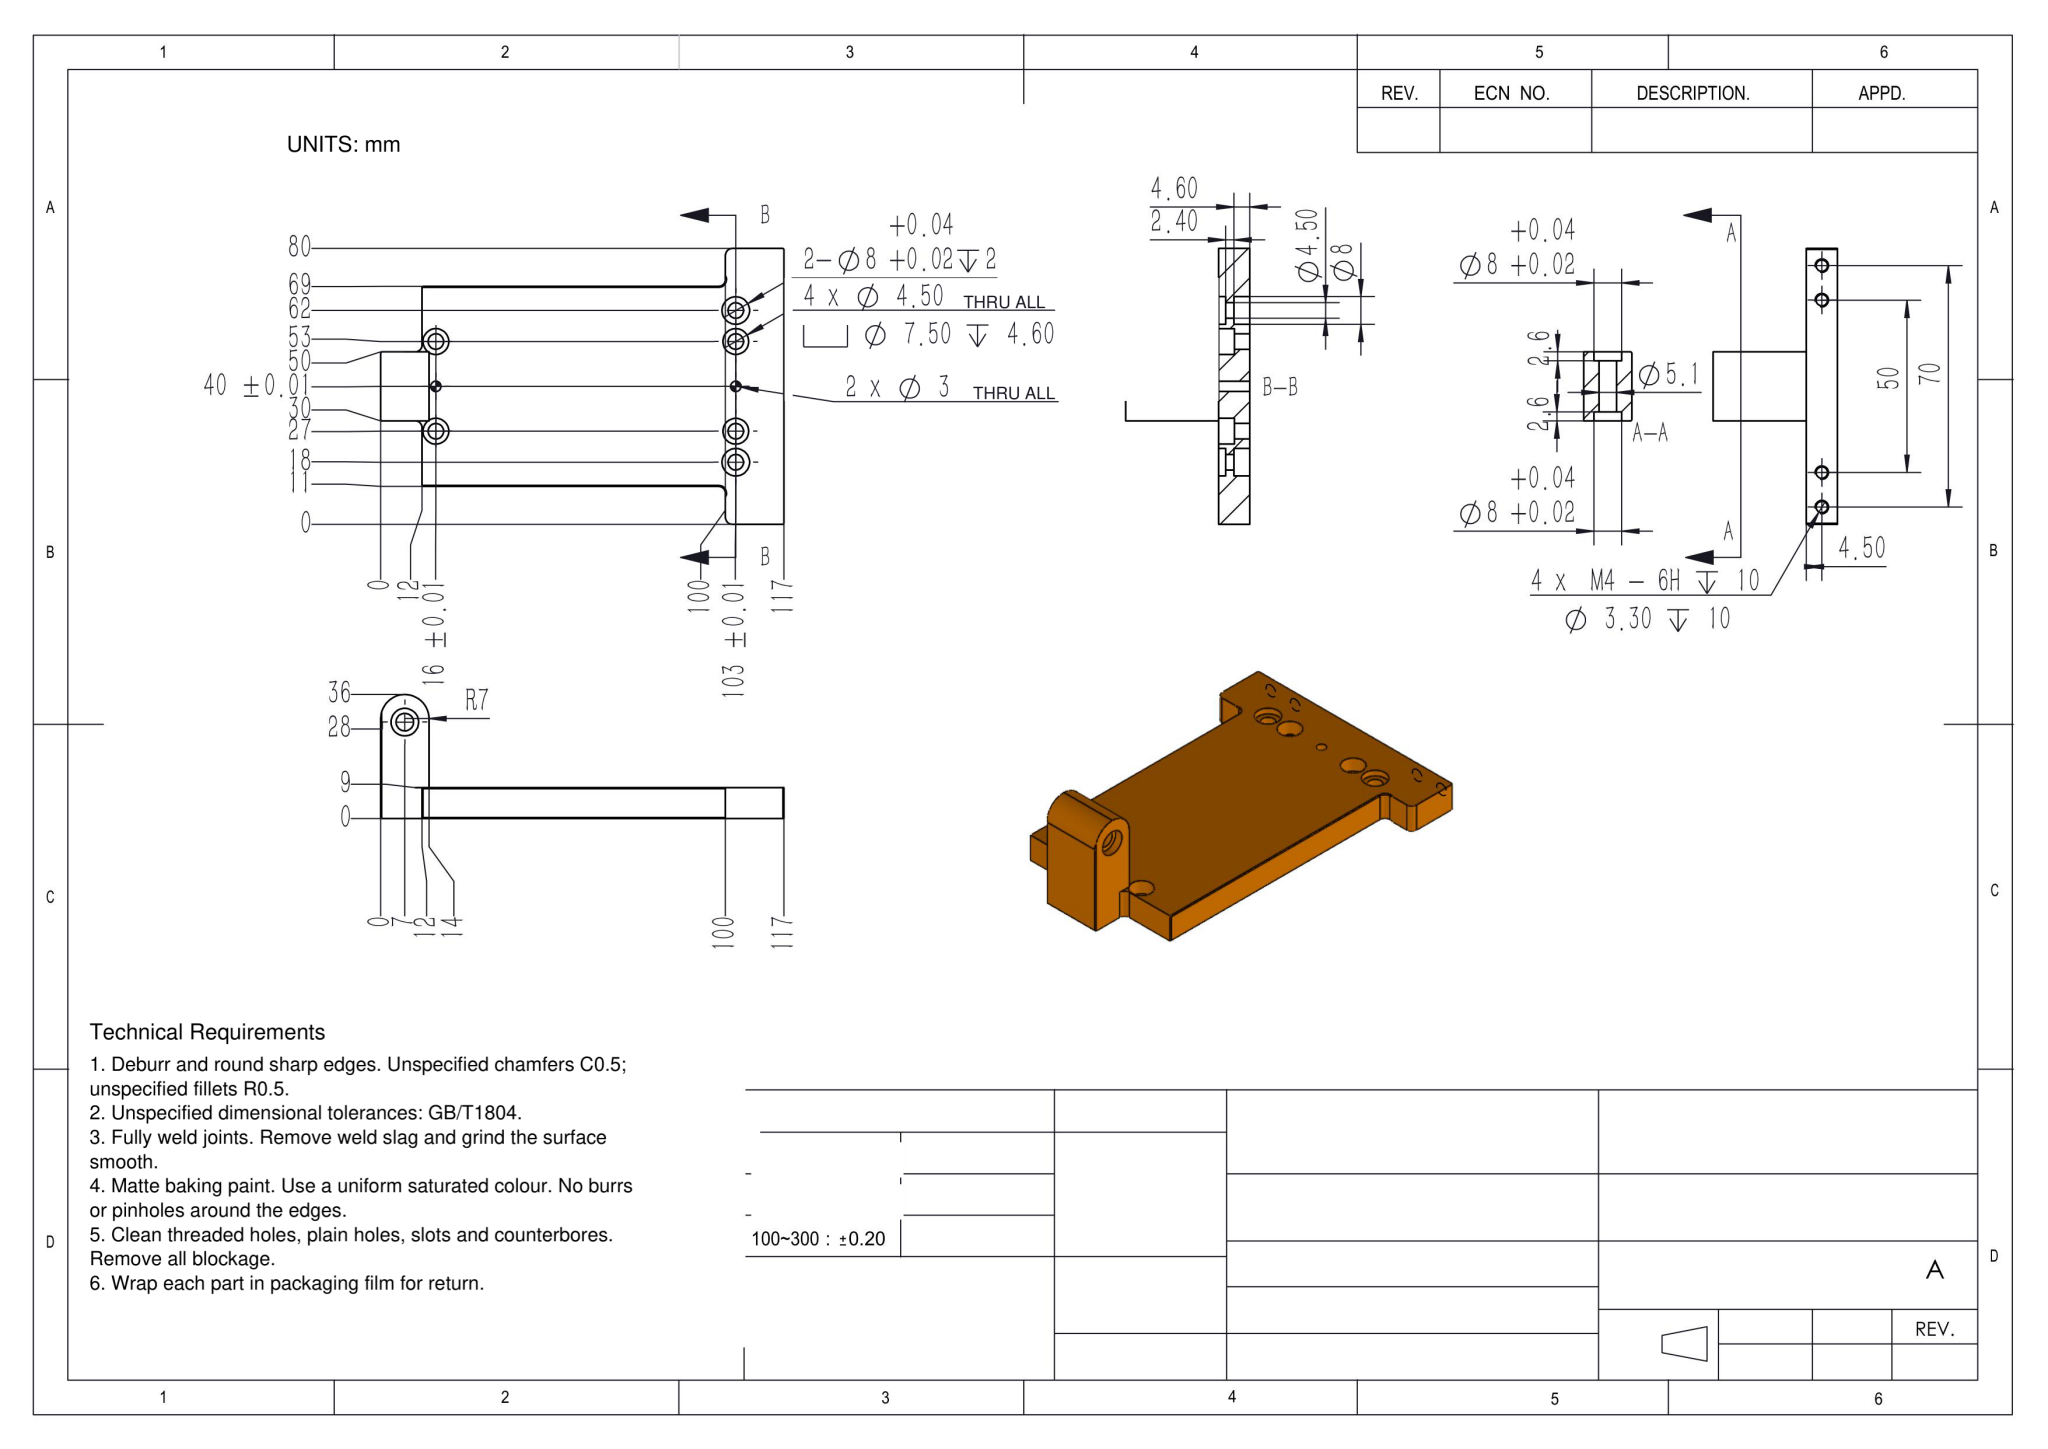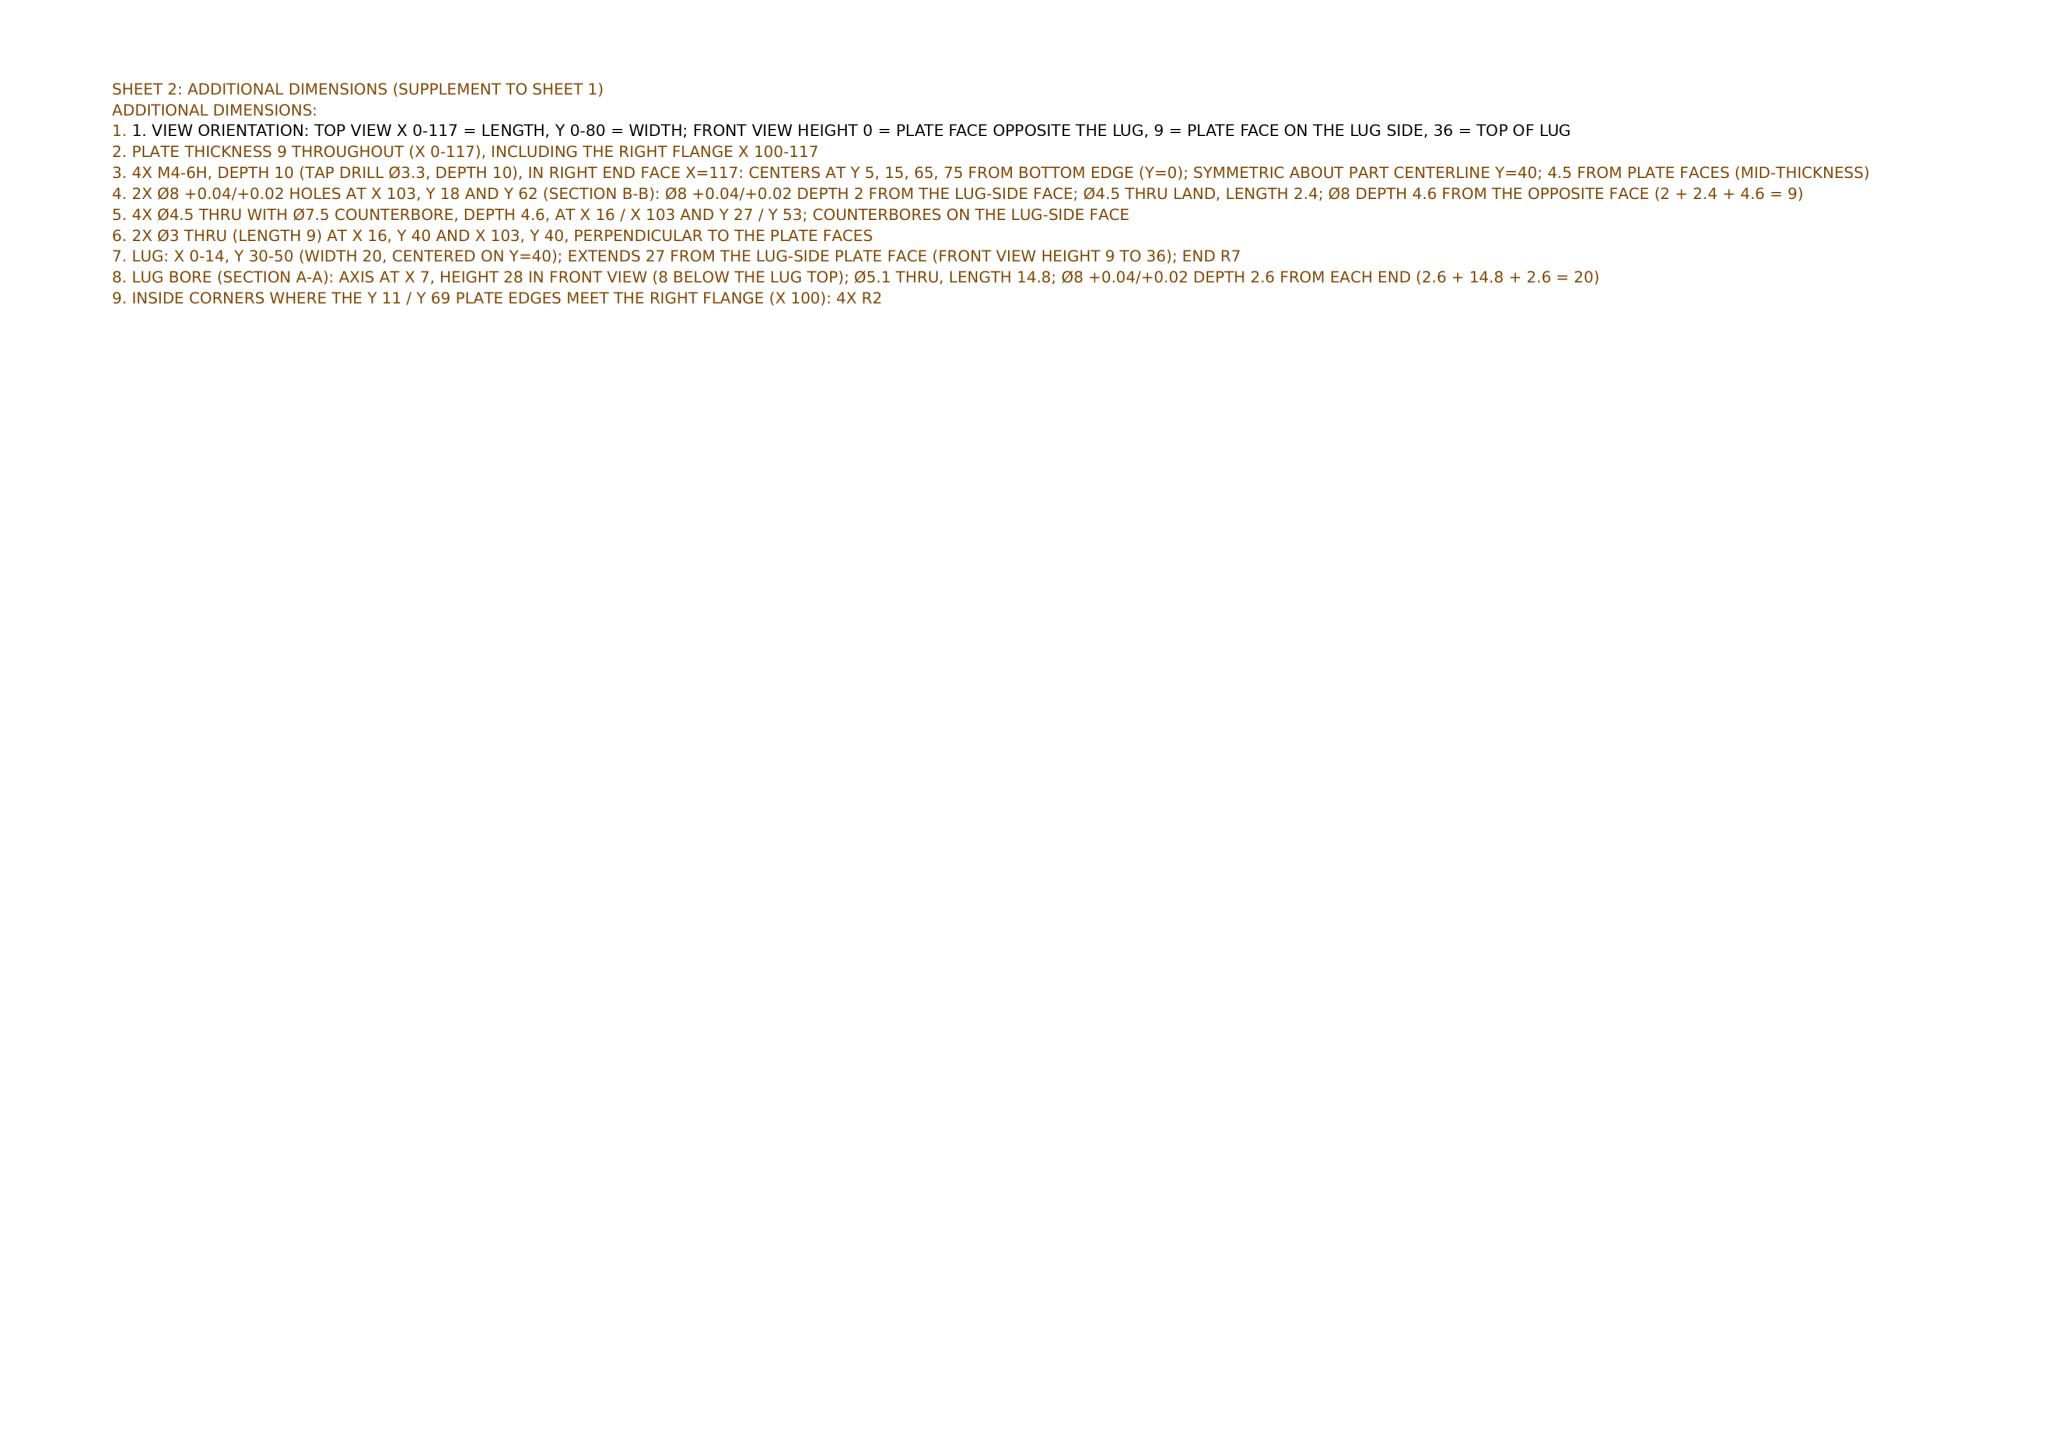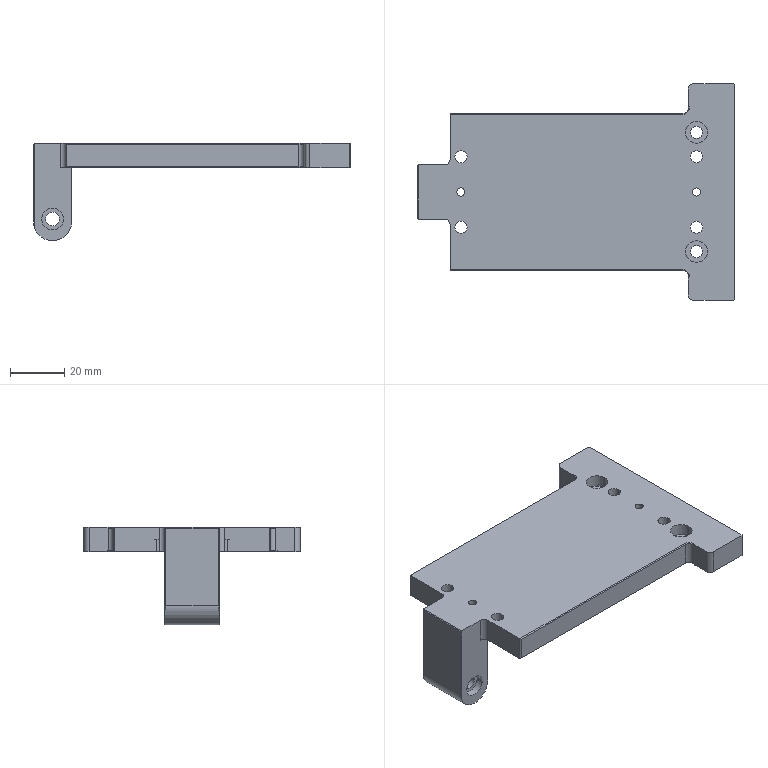Part | NX | mm | 1 solid | 106 faces | box 117 x 80 x 36 mm | volume 64592 mm3 | cylinder 54 | plane 38 | cone 14 | commonest cylinder face diameters 8 x12 4.5 x12 3.3 x8 7.5 x8 4 x6 3 x4 5.1 x2 14 x2